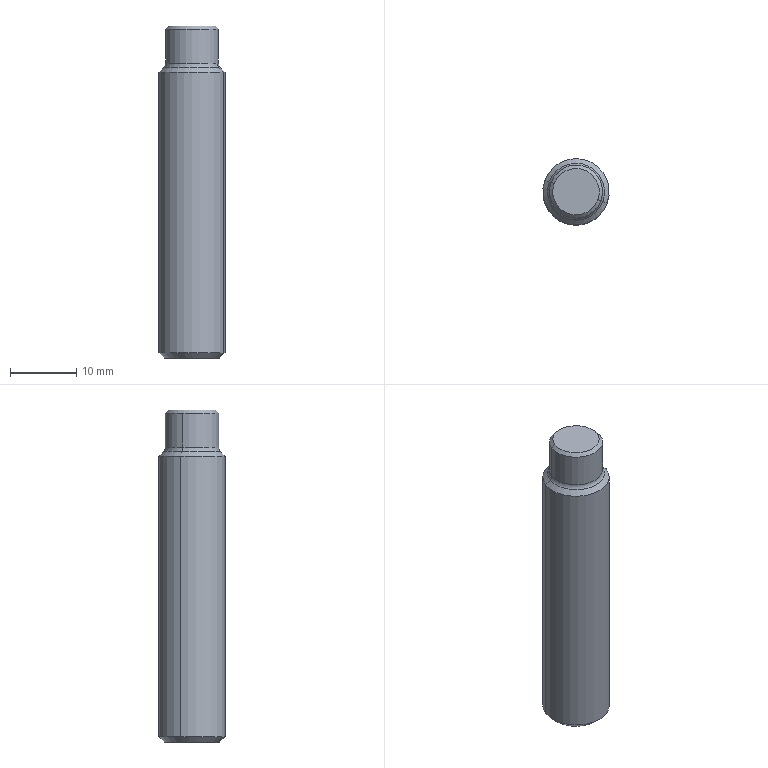Component | SolidWorks | MSSG10-50-2 | 1 solid | 28 faces | volume 3538 mm3 | plane 14 | cone 8 | cylinder 4 | torus 2 | commonest cylinder face diameters 10 x2 8 x2 | material S45C